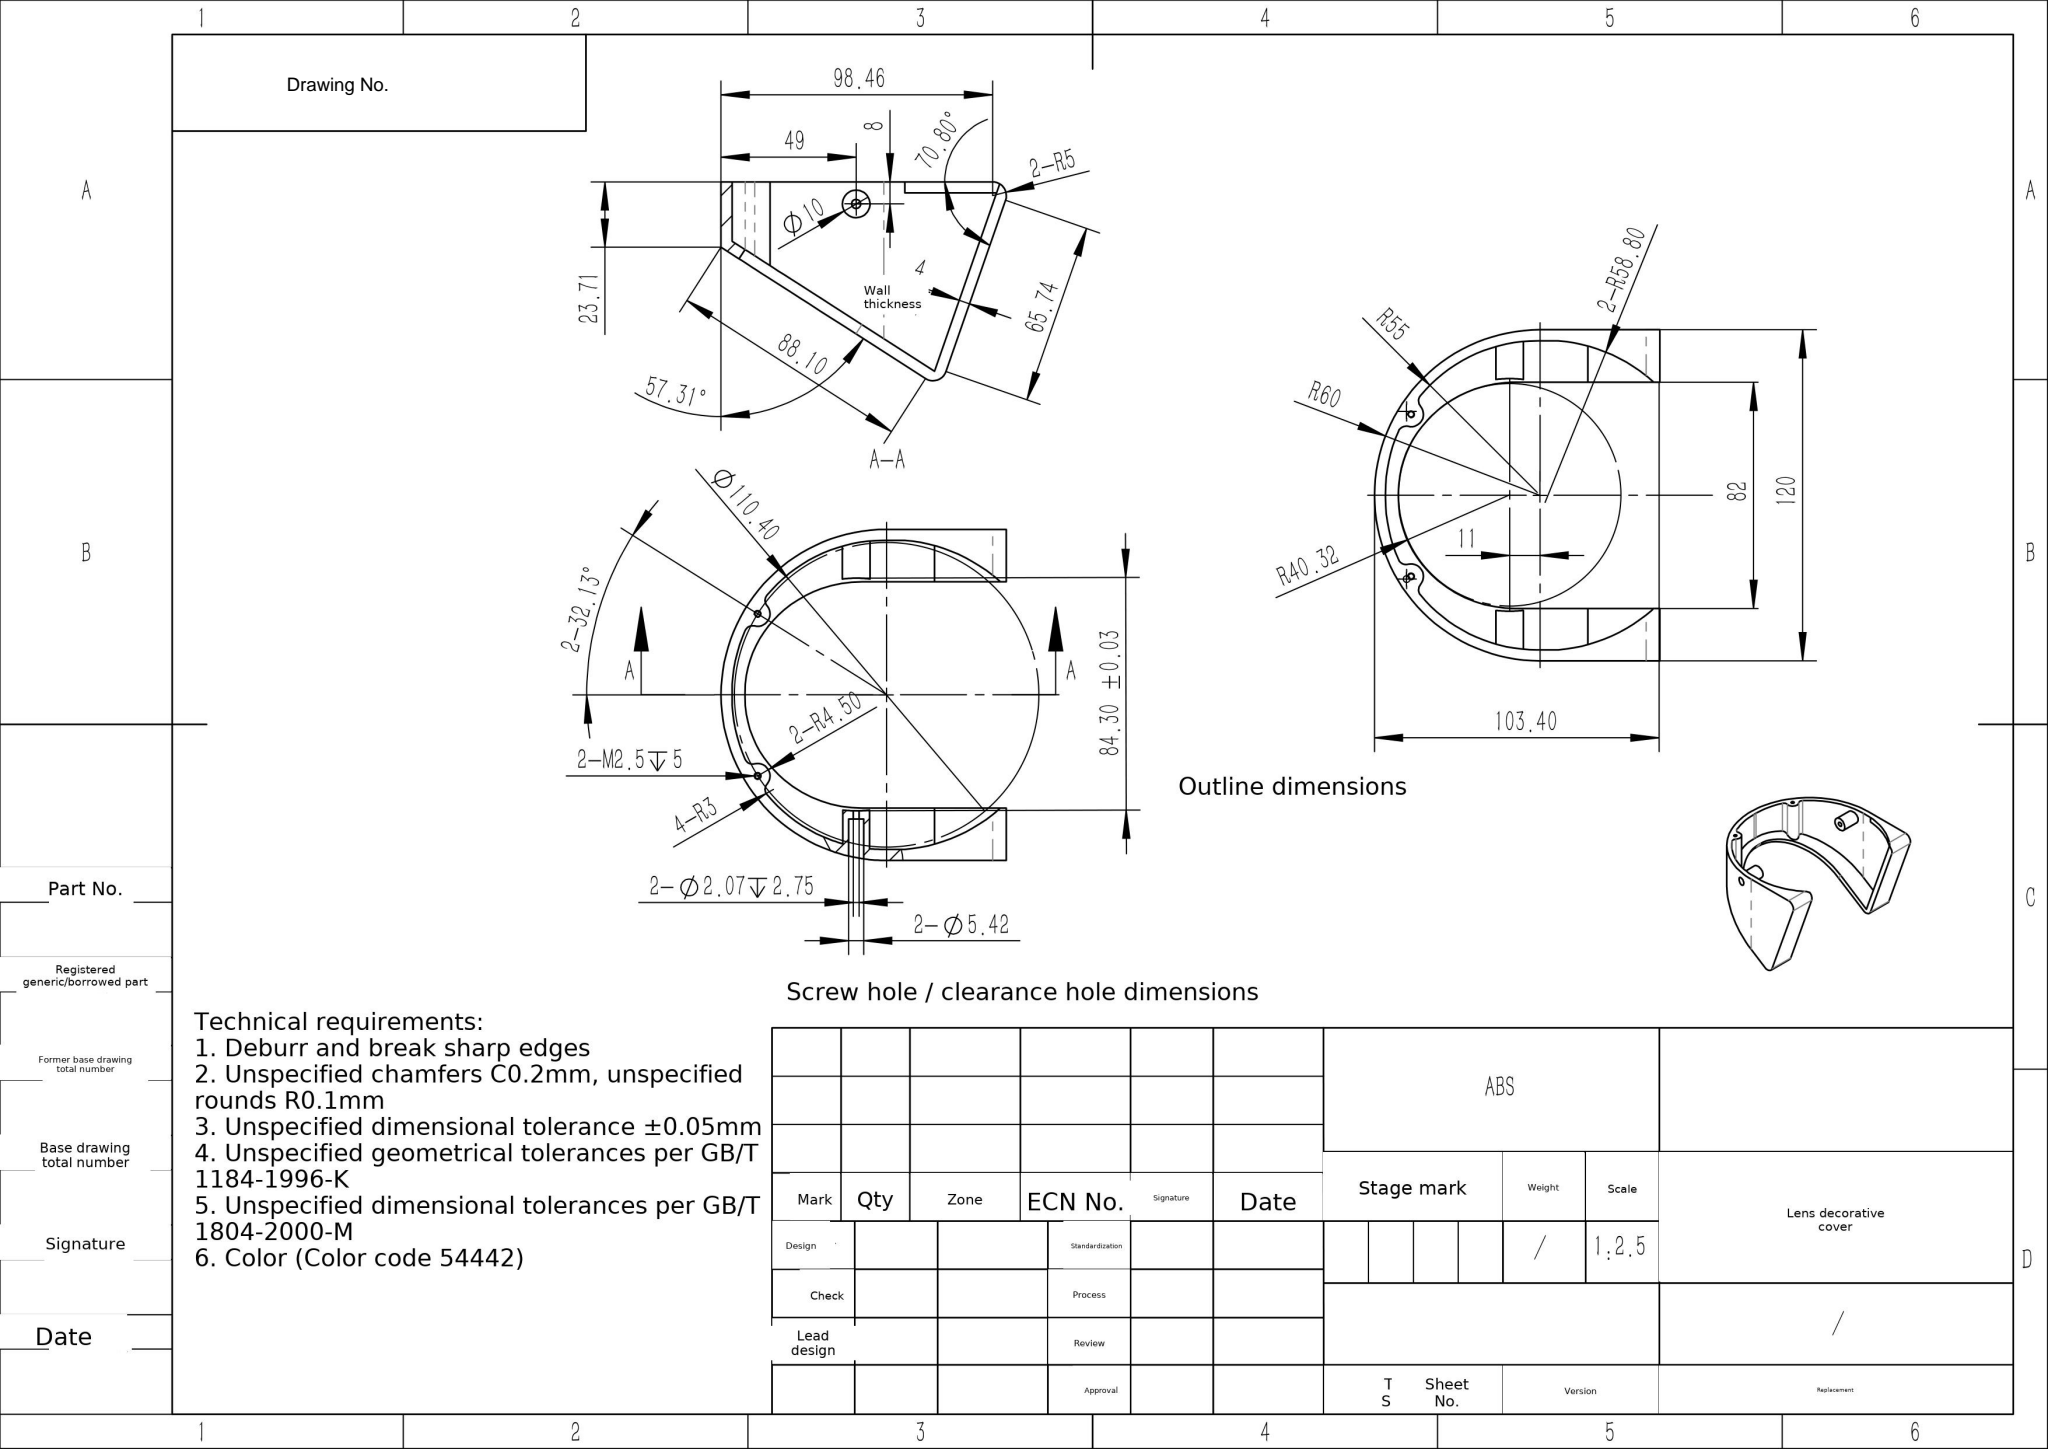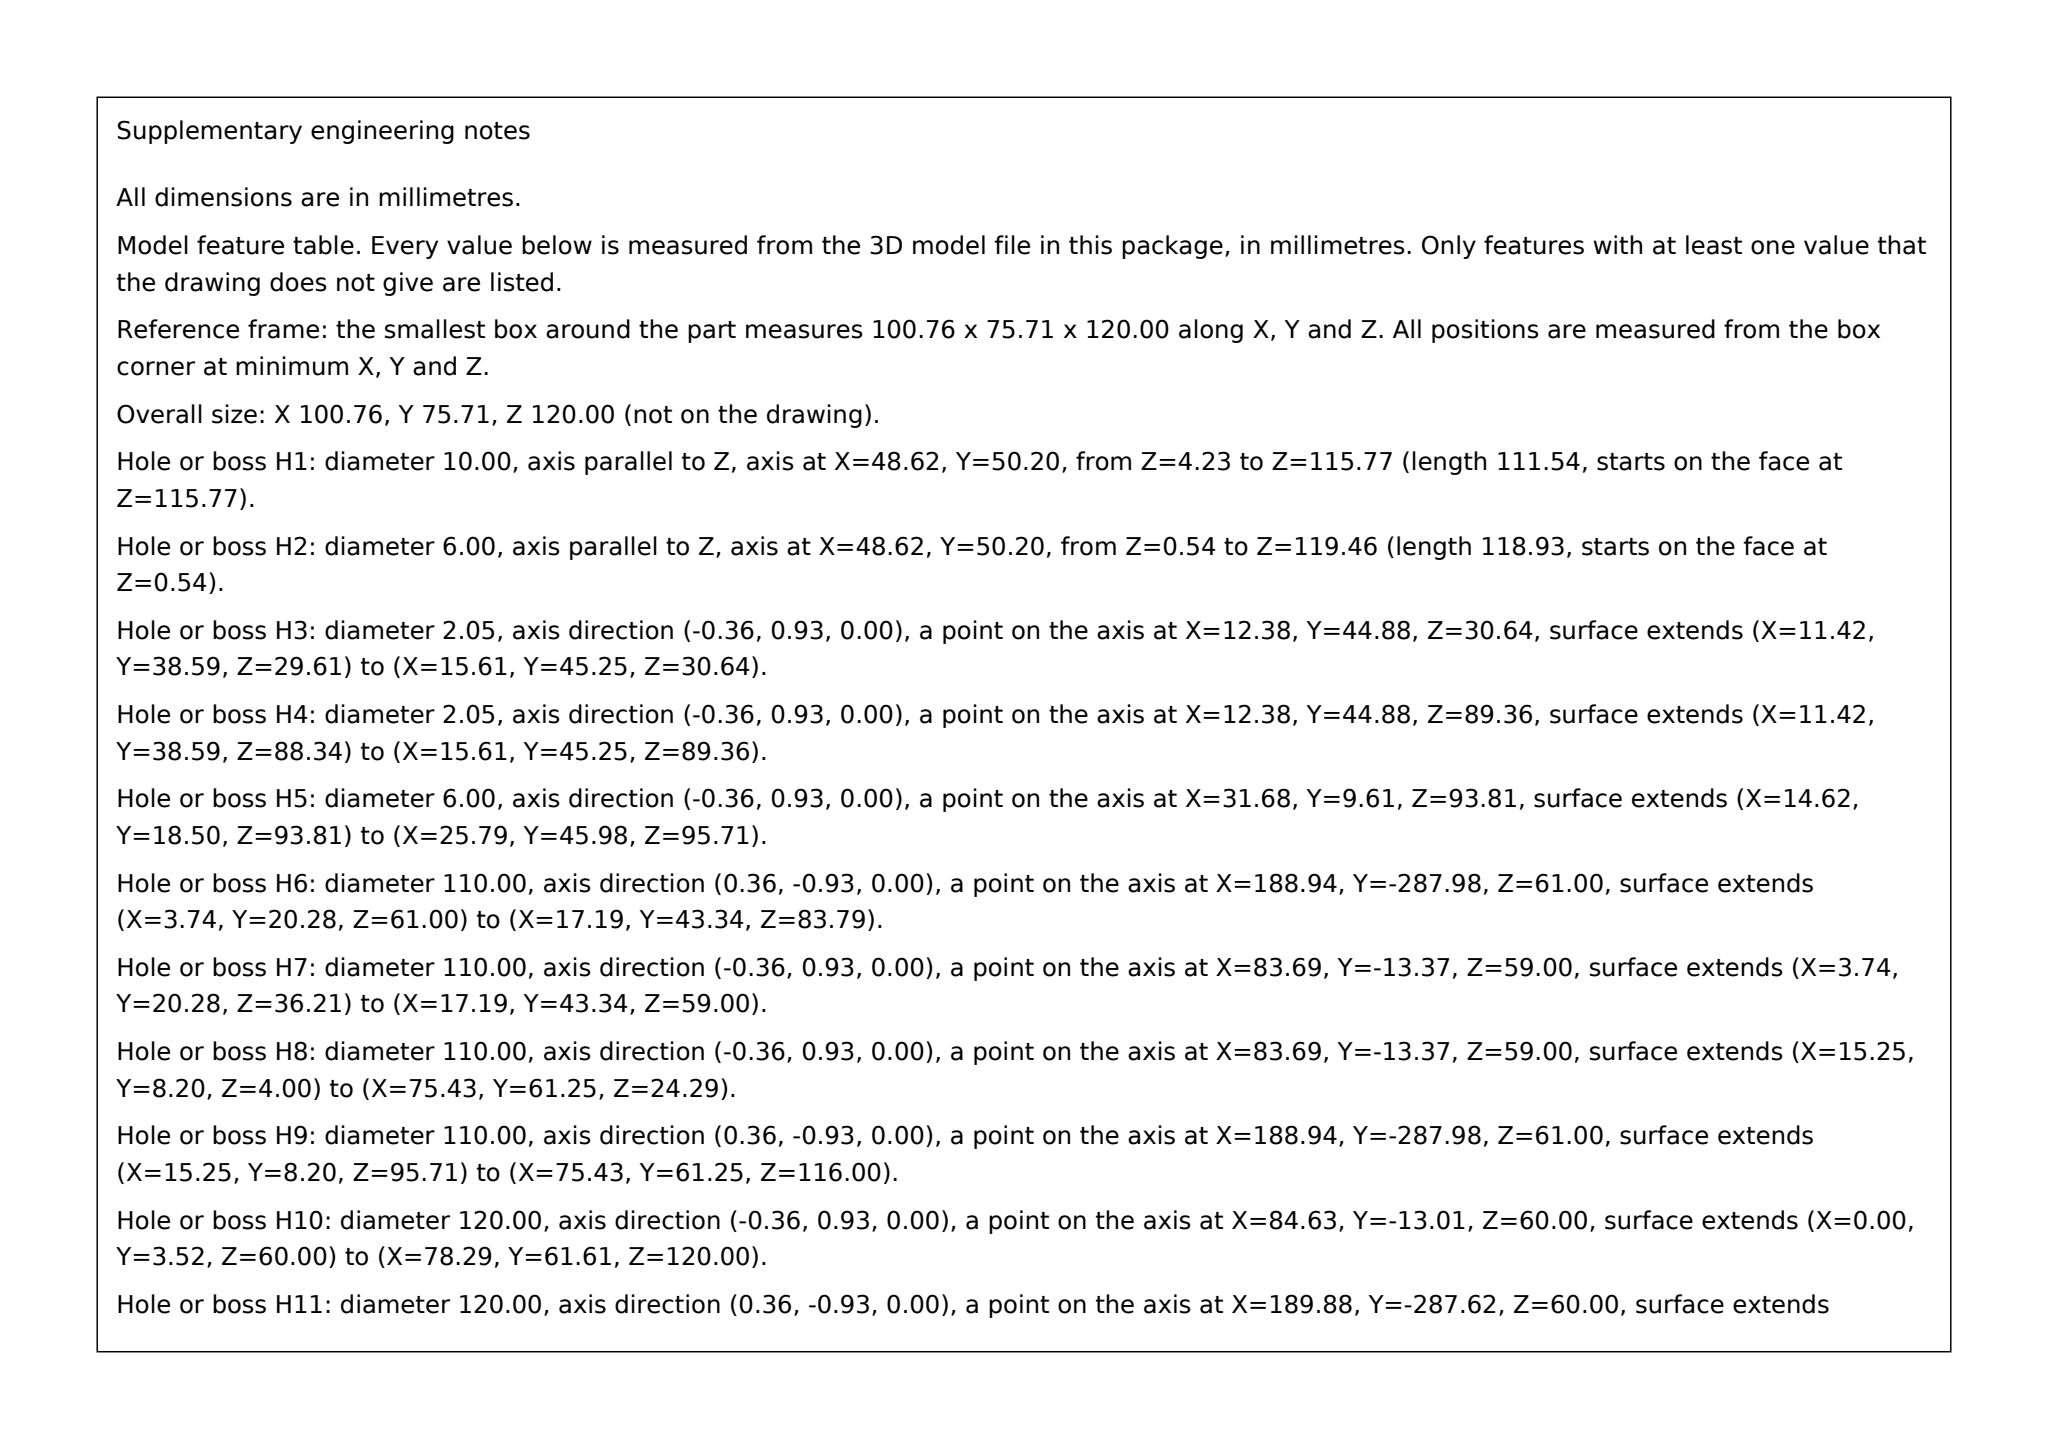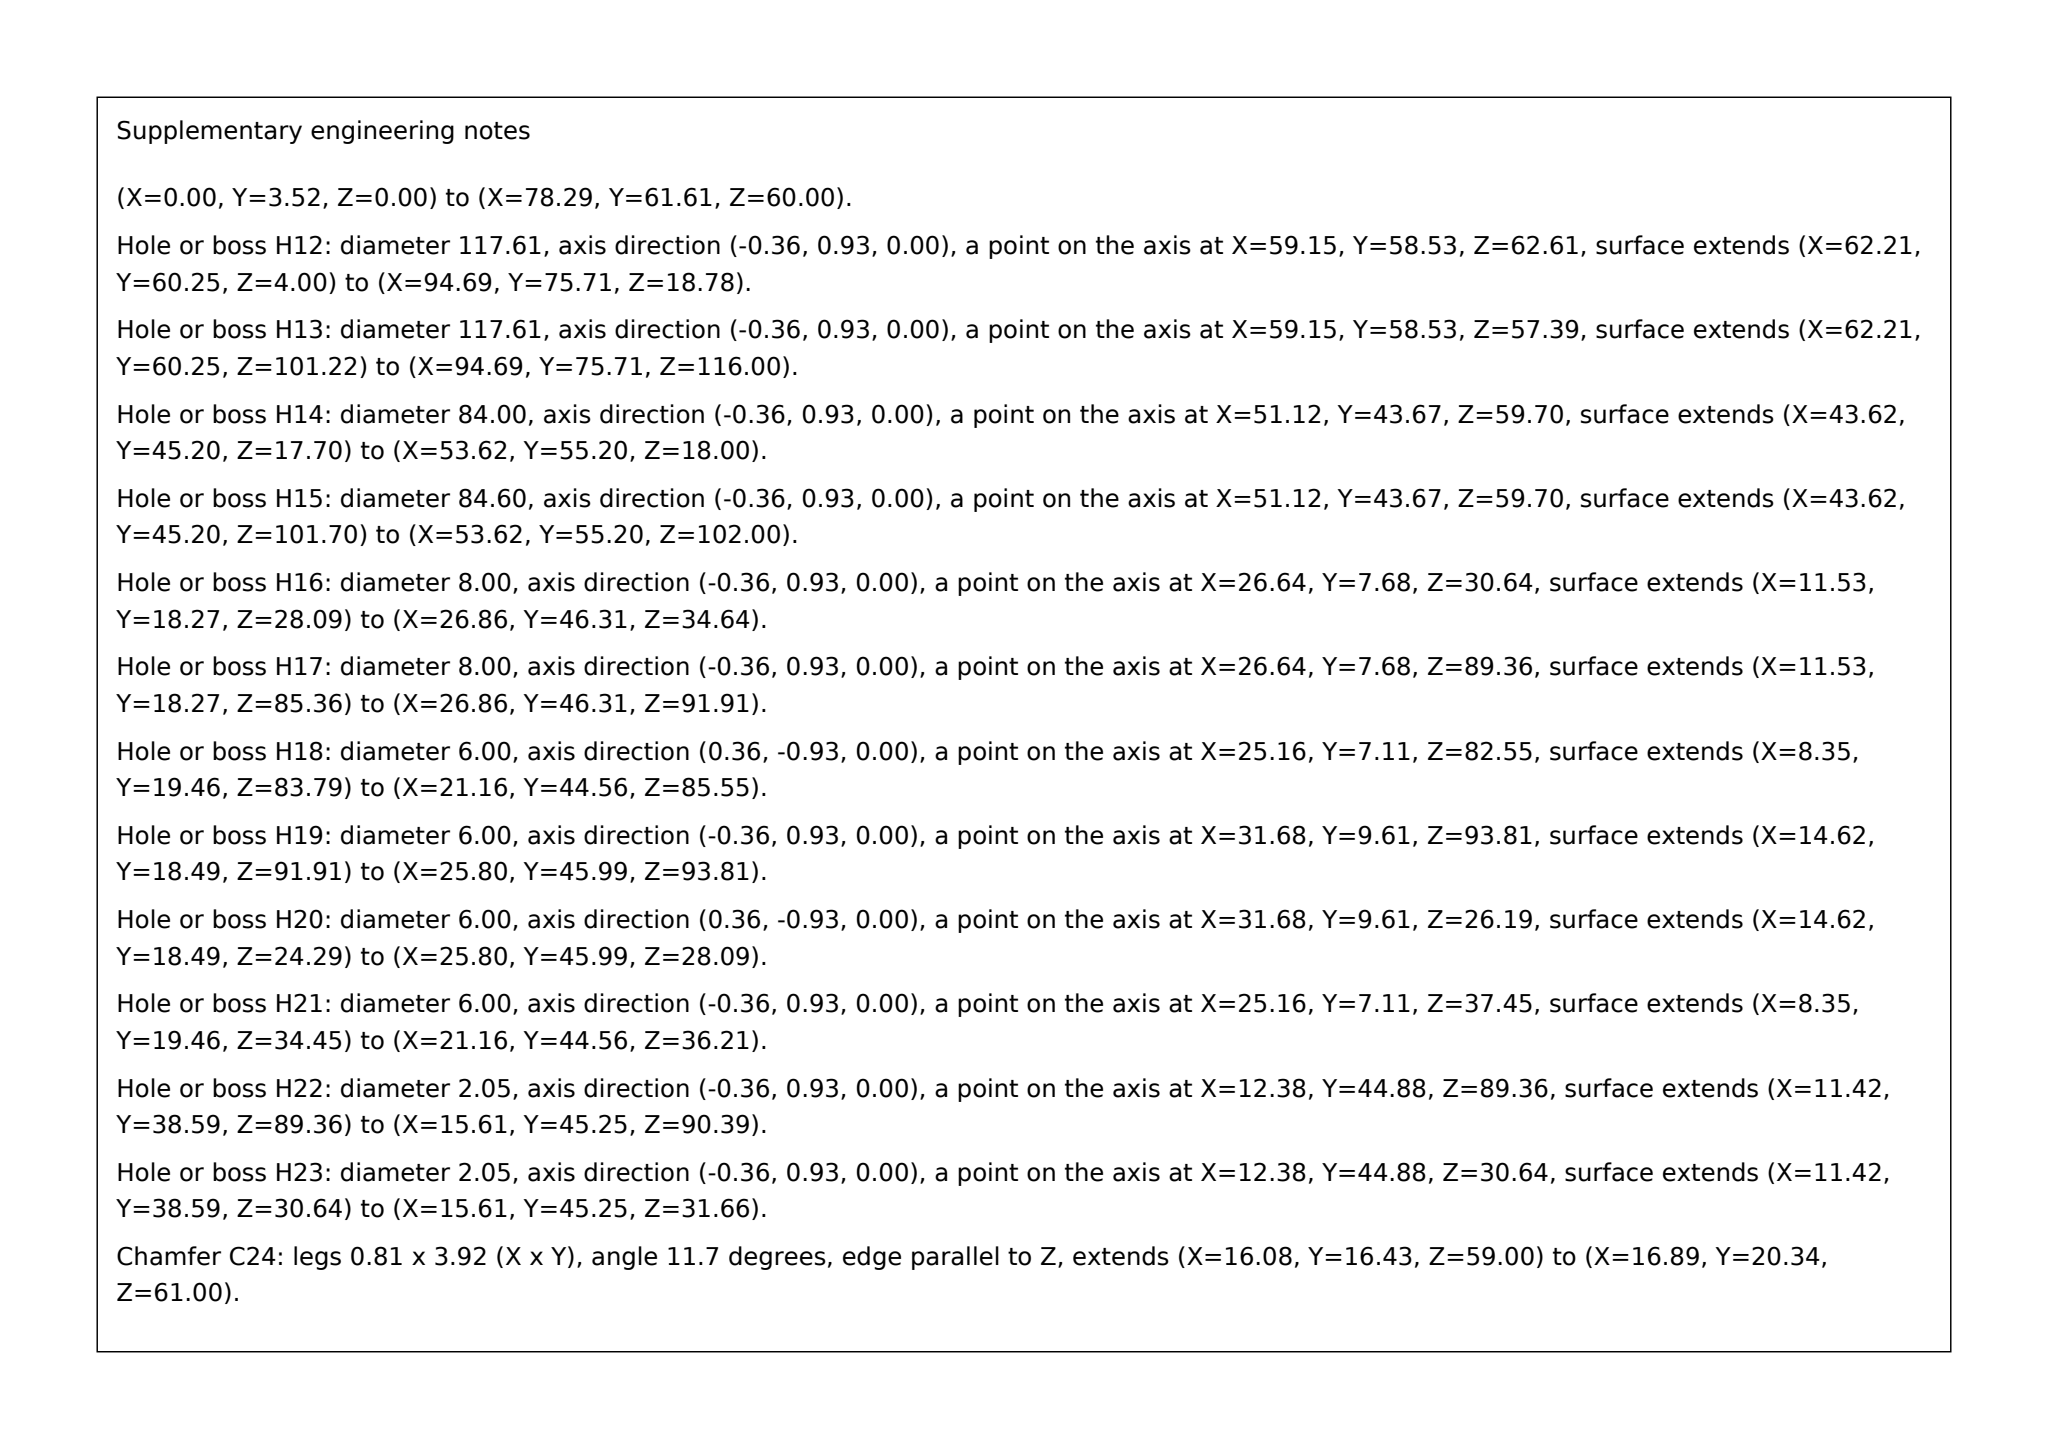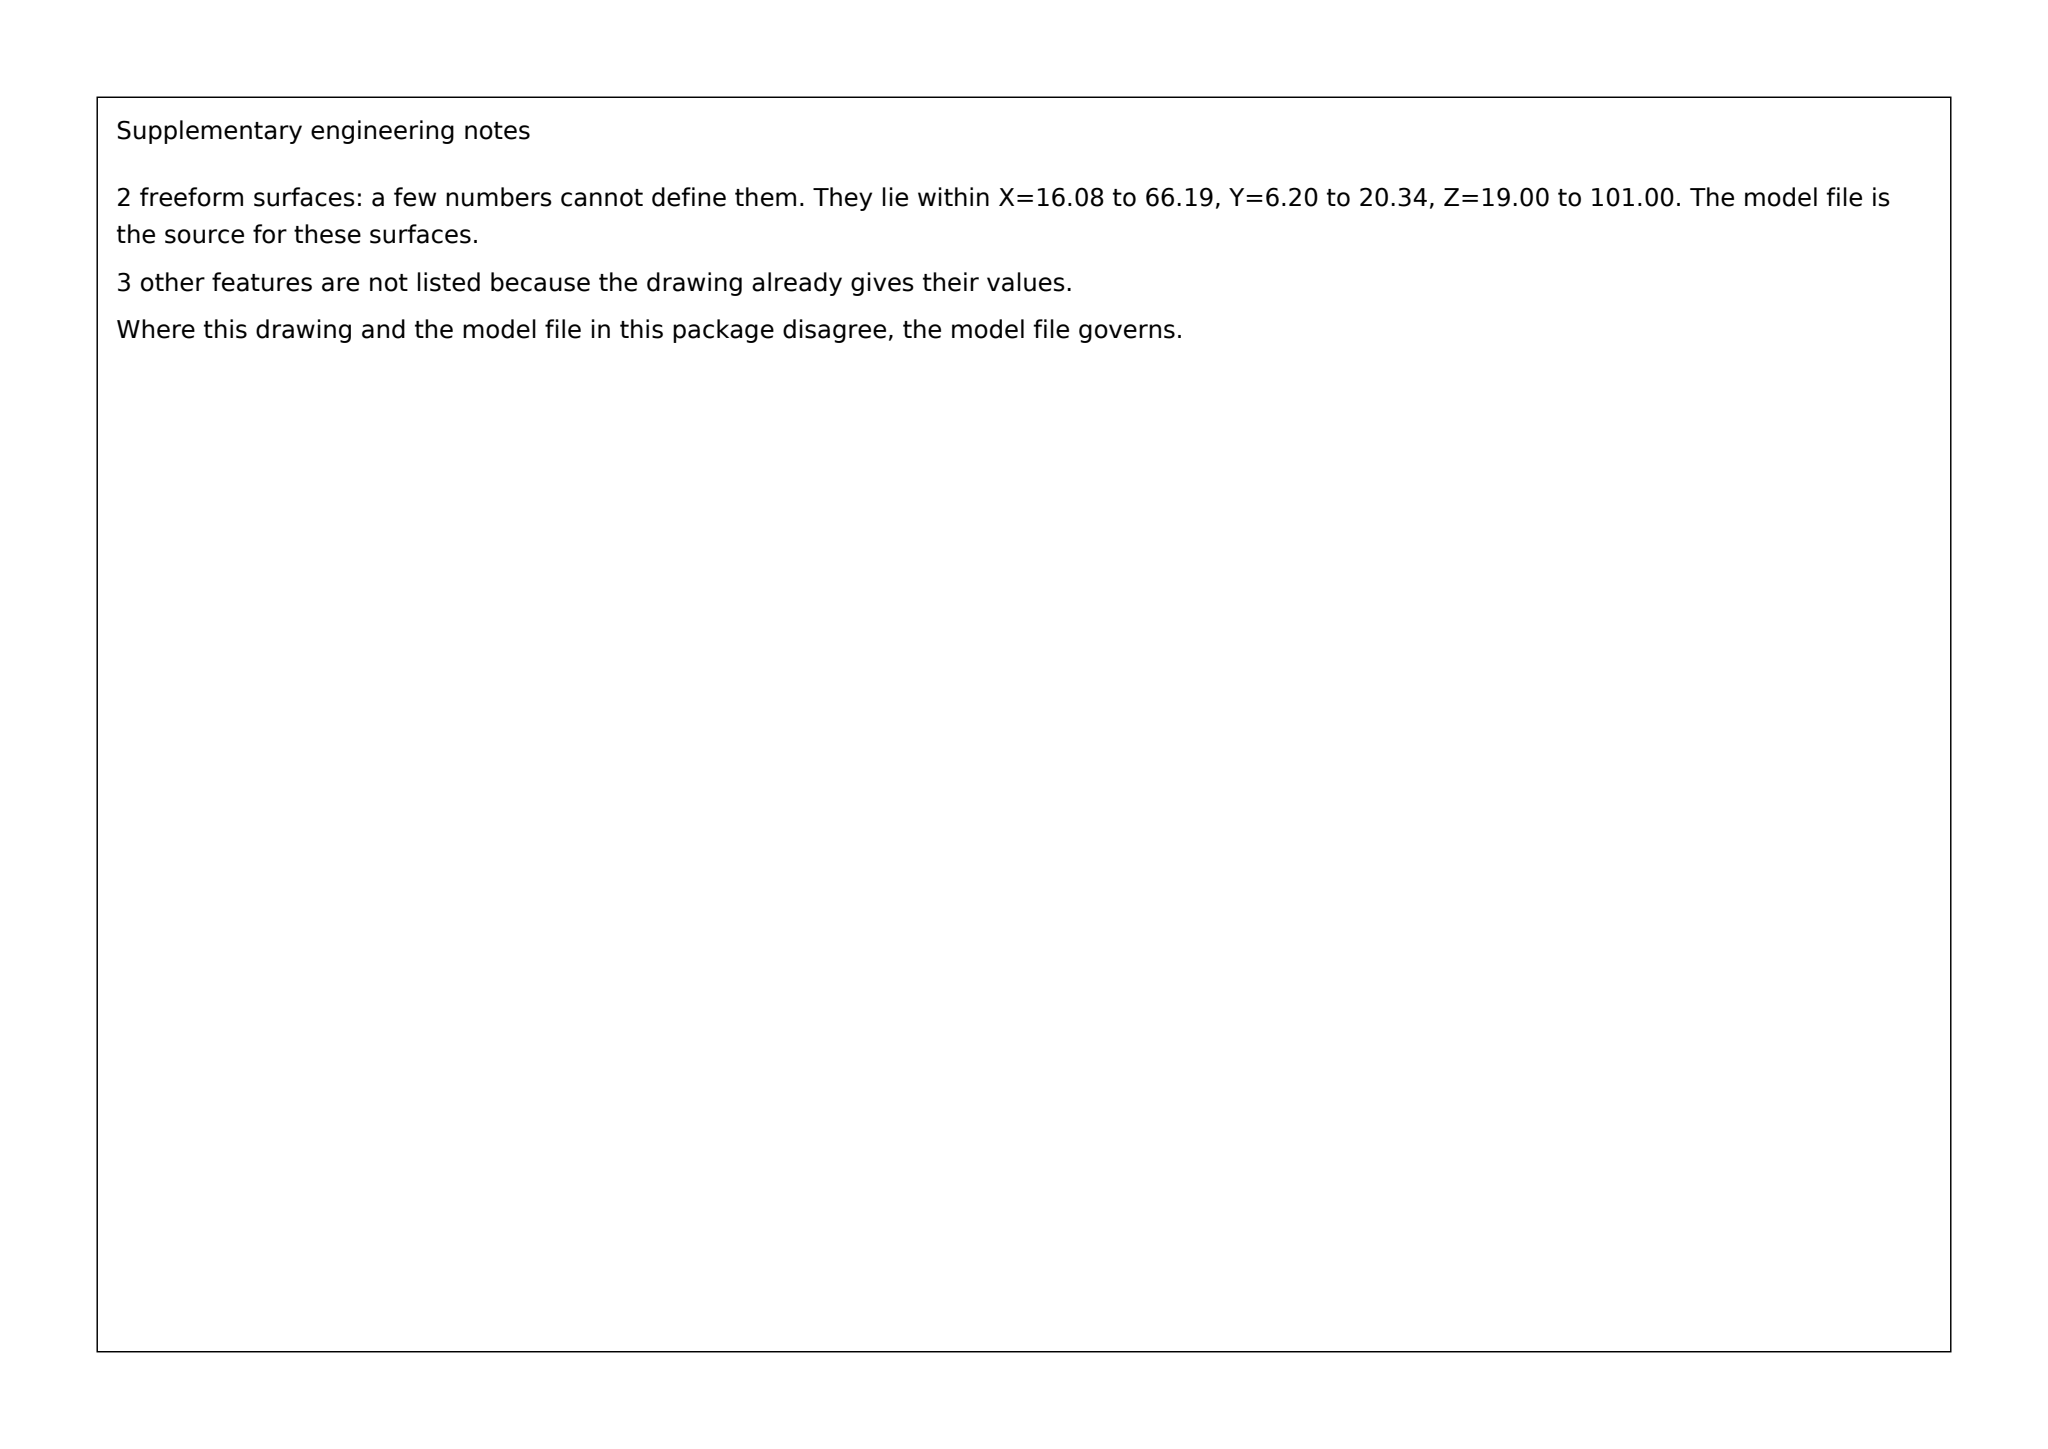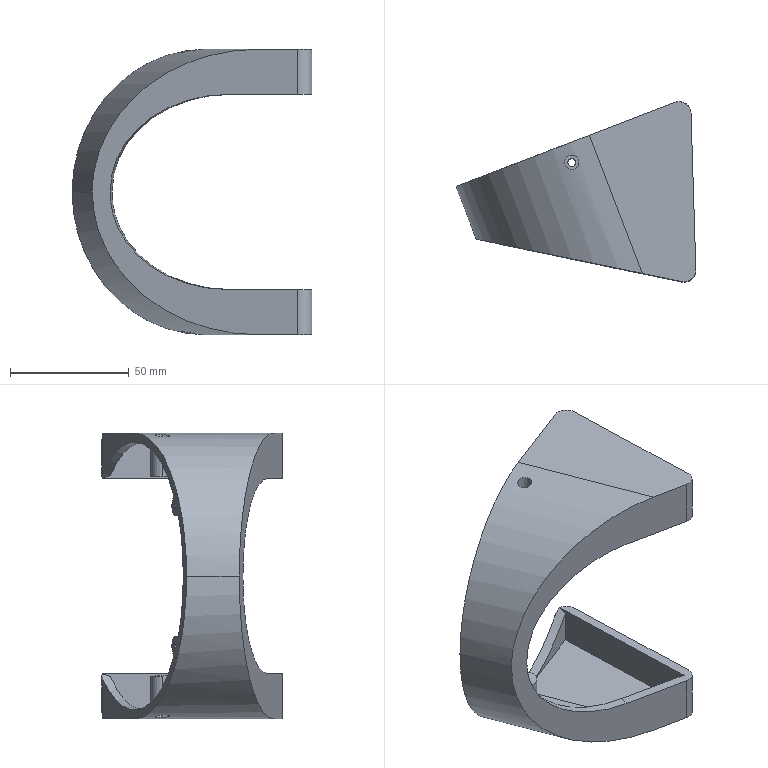Part | SolidWorks | mm | material ABS | 1 solid | 63 faces | box 100.76 x 75.71 x 120 mm | volume 66971 mm3 | cylinder 38 | plane 19 | cone 4 | spline 2 | commonest cylinder face diameters 6 x9 10 x9 2.05 x4 3.3 x4 110 x4 120 x2 117.608 x2 8 x2